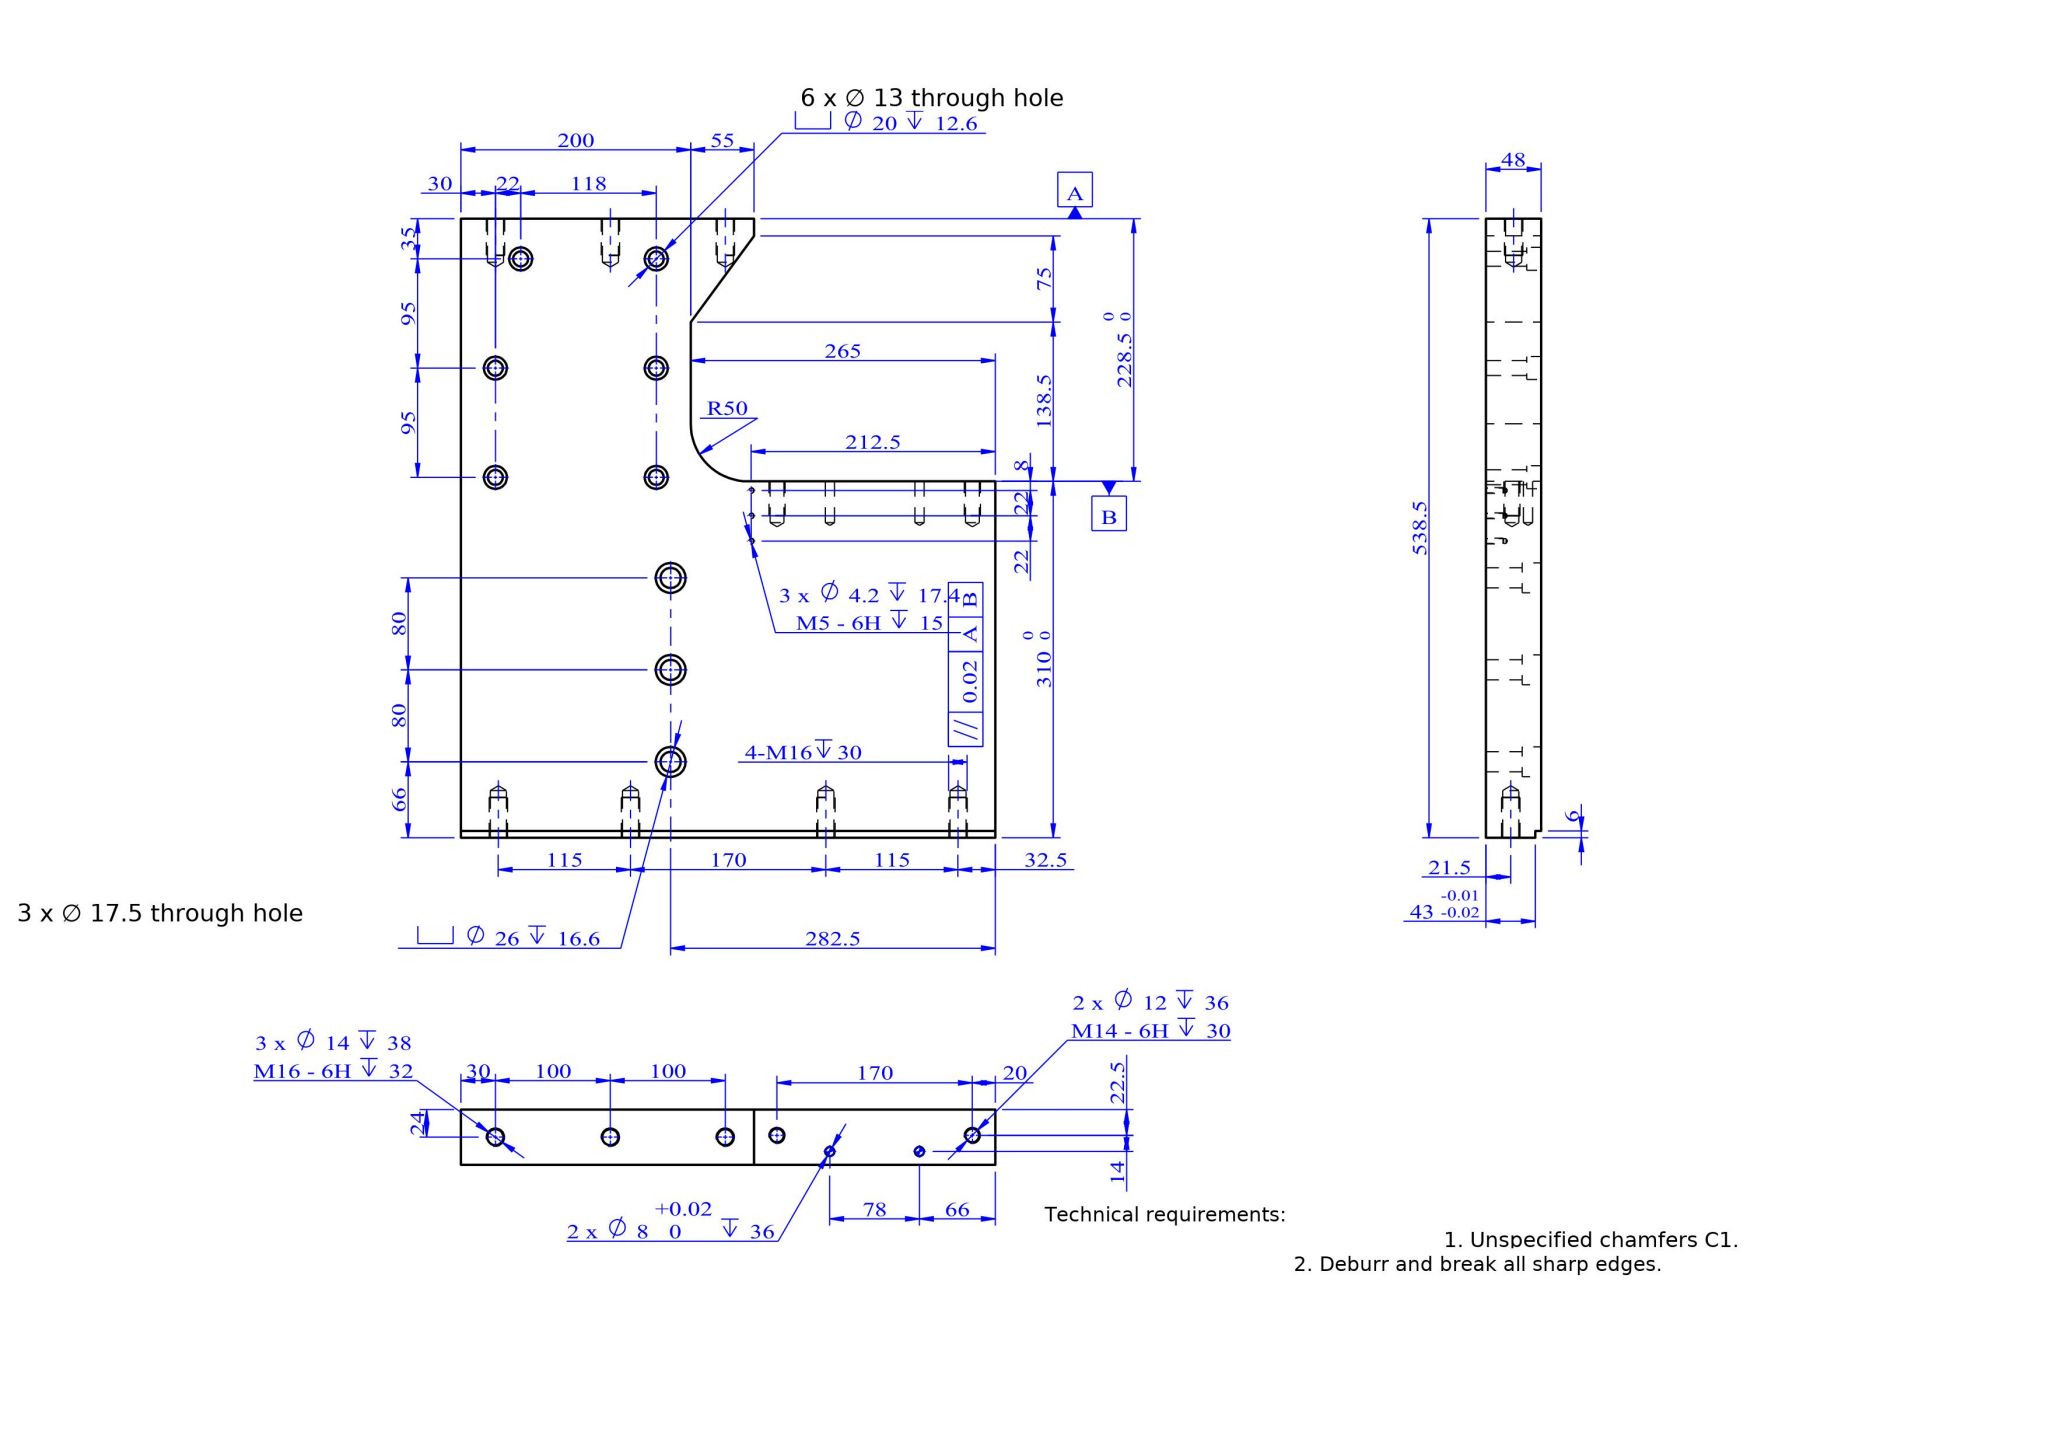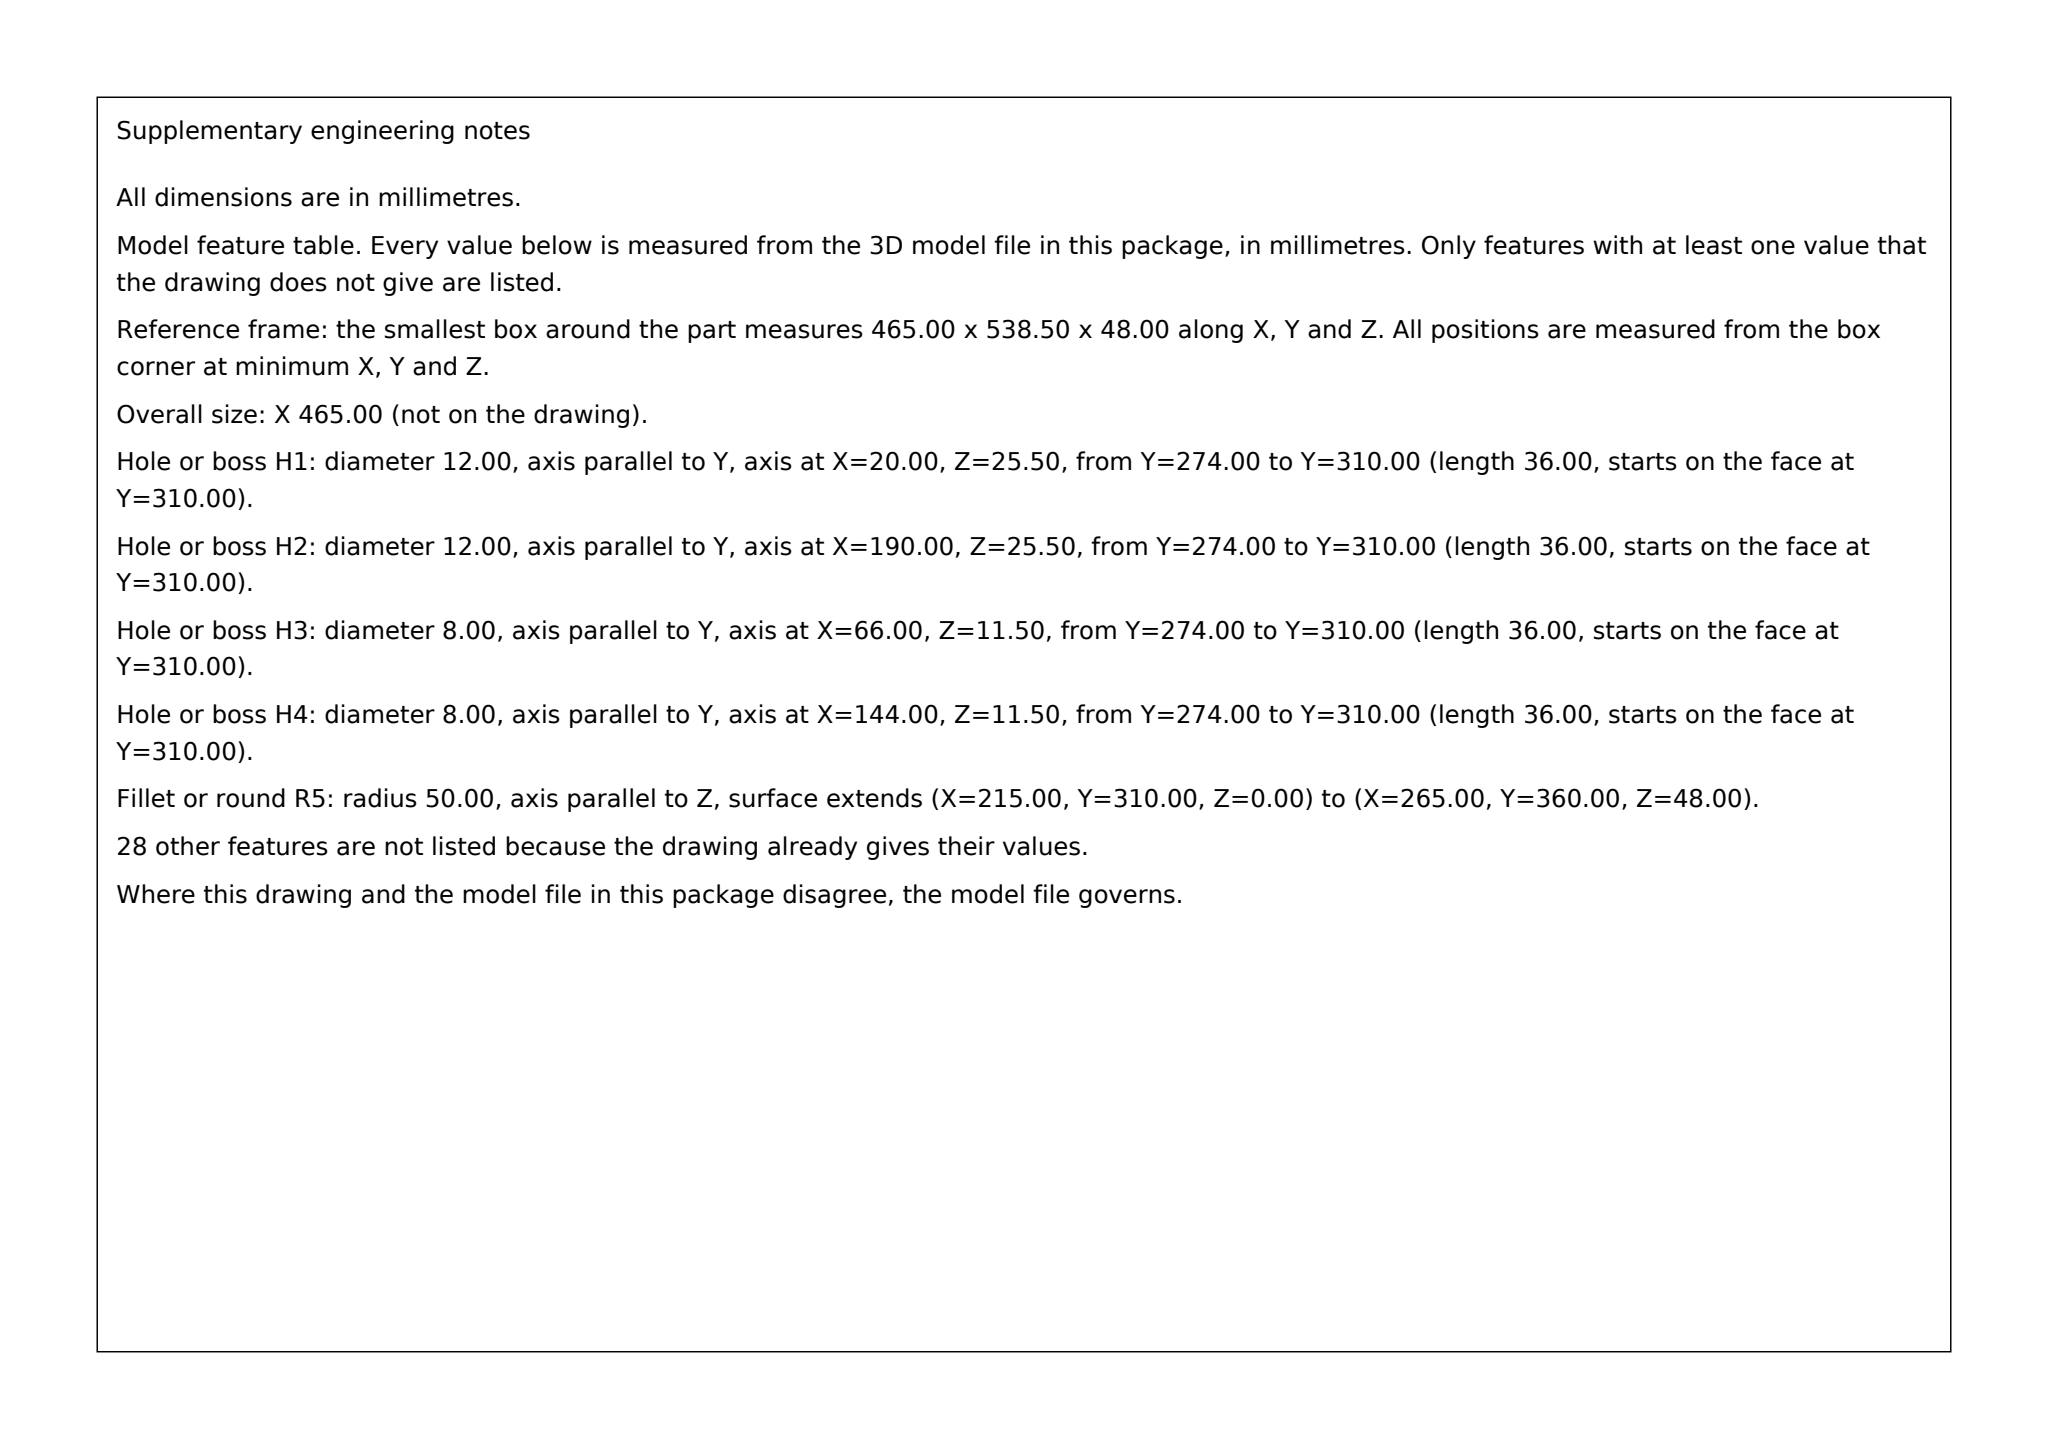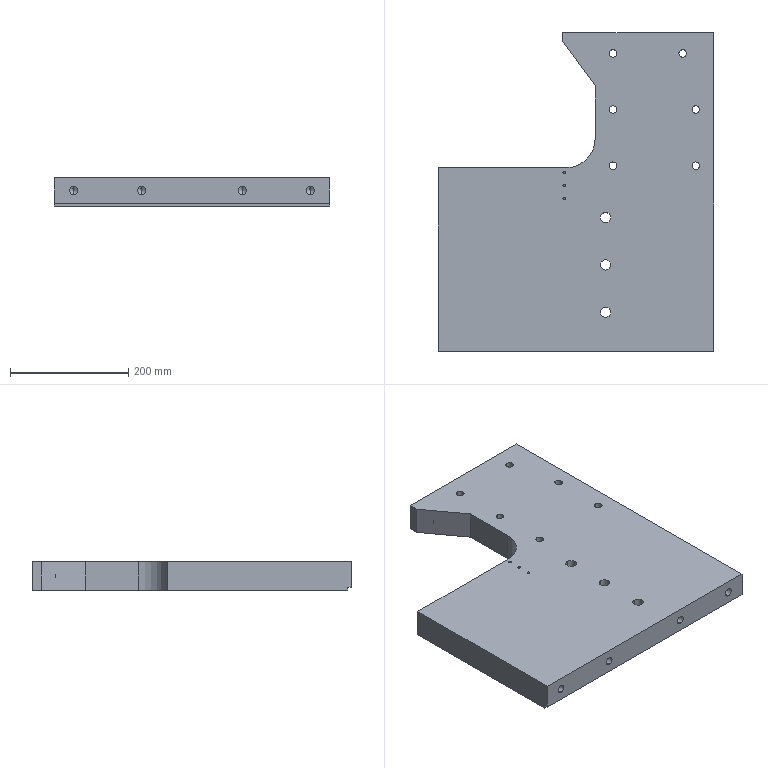Part | SolidWorks | mm | 1 solid | 114 faces | box 465 x 538.5 x 48 mm | volume 9105001 mm3 | cylinder 65 | cone 28 | plane 21 | commonest cylinder face diameters 14 x14 20 x12 13 x12 4.2 x6 26 x6 17.5 x6 8 x4 12 x4